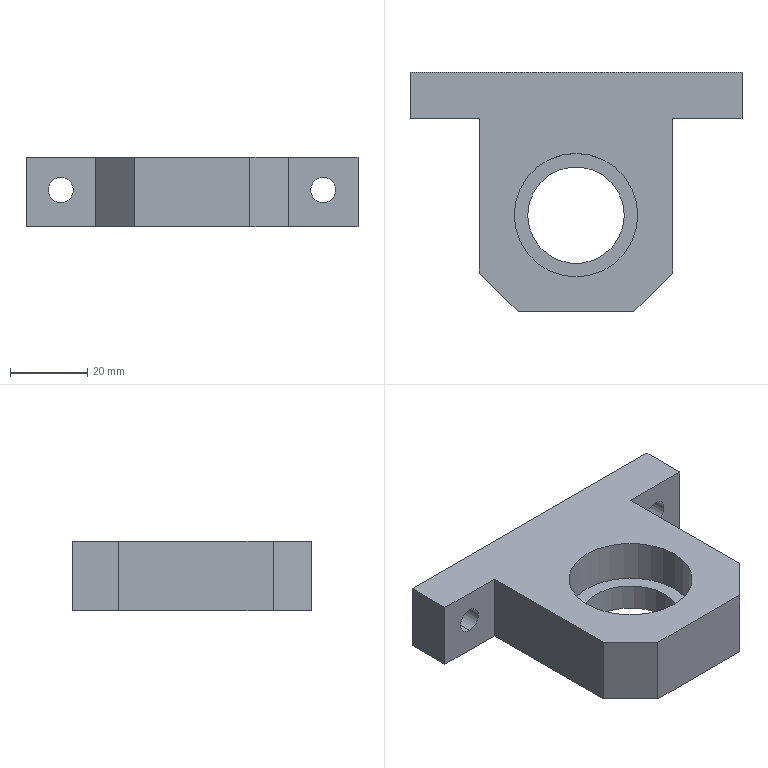Component | SolidWorks | --MA18S20041JR-SHuangGWBearingHousing1-1 | 1 solid | 21 faces | box 86 x 62 x 18 mm | volume 48697 mm3 | plane 13 | cylinder 8 | commonest cylinder face diameters 6.5 x4 25 x2 32 x2
build123d program:
from build123d import *

# Parameters (mm, degrees)
SKETCH1_W                  = 50
SKETCH1_H                  = 50
BOSS_EXTRUDE1_DEPTH        = 18
SKETCH2_W                  = 86
SKETCH2_H                  = 18
BOSS_EXTRUDE2_DEPTH        = 12
CHAMFER1_SIZE              = 10
SKETCH3_R                  = 16
CUT_EXTRUDE1_DEPTH         = 11
SKETCH4_R                  = 12.5
CUT_EXTRUDE2_DEPTH         = 86.118
F_6_5_6_5_DIAMETER_HOLE1_D = 6.5


with BuildPart() as part:
    # Sketch1 → Boss-Extrude1 (new body)
    with BuildSketch(Plane.XY):
        with Locations((25, 25)):
            Rectangle(SKETCH1_W, SKETCH1_H)
    extrude(amount=BOSS_EXTRUDE1_DEPTH)

    # Sketch2 → Boss-Extrude2 (add)
    with BuildSketch(Plane.XZ):
        with Locations((25, 9)):
            Rectangle(SKETCH2_W, SKETCH2_H)
    extrude(amount=BOSS_EXTRUDE2_DEPTH)

    # Chamfer1
    chamfer1_edges = [part.edges().sort_by_distance(p)[0] for p in [
        (0, 50, 9),
        (50, 50, 9),
    ]]
    chamfer(chamfer1_edges, length=CHAMFER1_SIZE)

    # Sketch3 → Cut-Extrude1 (cut)
    with BuildSketch(Plane.XY.offset(18)):
        with Locations((25, 25)):
            Circle(SKETCH3_R)
    extrude(amount=-CUT_EXTRUDE1_DEPTH, mode=Mode.SUBTRACT)

    # Sketch4 → Cut-Extrude2 (cut, through all)
    with BuildSketch(Plane.XY.offset(7)):
        with Locations((25, 25)):
            Circle(SKETCH4_R)
    extrude(amount=-CUT_EXTRUDE2_DEPTH, mode=Mode.SUBTRACT)

    # 6.5 _6.5_ Diameter Hole1 (through all)
    with Locations(Plane(origin=(0, 0, 0), x_dir=(-1, 0, 0), z_dir=(0, 1, 0))):
        with Locations((-59, 9.5), (9, 9.5)):
            Hole(F_6_5_6_5_DIAMETER_HOLE1_D / 2)


solid = part.part

# Placed as in the assembly
solid = solid.moved(Location((97.885, -8.301, 1), (0, 0, 180)))
STEP:
#1=COLOUR_RGB('',0.7922,0.8196,0.9333);
#2=FILL_AREA_STYLE_COLOUR('',#1);
#3=FILL_AREA_STYLE('',(#2));
#4=SURFACE_STYLE_FILL_AREA(#3);
#5=SURFACE_SIDE_STYLE('',(#4));
#6=SURFACE_STYLE_USAGE(.BOTH.,#5);
#7=PRESENTATION_STYLE_ASSIGNMENT((#6));
#8=CARTESIAN_POINT('',(1.531,0.1456,0.2854));
#9=VERTEX_POINT('',#8);
#10=CARTESIAN_POINT('',(1.531,0.1456,0.5413));
#11=VERTEX_POINT('',#10);
#12=CARTESIAN_POINT('',(1.531,0.1456,0.4134));
#13=DIRECTION('',(-0.,-1.,0.));
#14=DIRECTION('',(0.,0.,1.));
#15=AXIS2_PLACEMENT_3D('',#12,#13,#14);
#16=CIRCLE('',#15,0.128);
#17=EDGE_CURVE('',#9,#11,#16,.T.);
#18=ORIENTED_EDGE('',*,*,#17,.F.);
#19=CARTESIAN_POINT('',(1.531,-0.3268,0.2854));
#20=VERTEX_POINT('',#19);
#21=CARTESIAN_POINT('',(1.531,-0.3268,0.2854));
#22=DIRECTION('',(-0.,-1.,0.));
#23=VECTOR('',#22,39.37);
#24=LINE('',#21,#23);
#25=EDGE_CURVE('',#9,#20,#24,.T.);
#26=ORIENTED_EDGE('',*,*,#25,.T.);
#27=CARTESIAN_POINT('',(1.531,-0.3268,0.5413));
#28=VERTEX_POINT('',#27);
#29=CARTESIAN_POINT('',(1.531,-0.3268,0.4134));
#30=DIRECTION('',(-0.,-1.,0.));
#31=DIRECTION('',(0.,0.,1.));
#32=AXIS2_PLACEMENT_3D('',#29,#30,#31);
#33=CIRCLE('',#32,0.128);
#34=EDGE_CURVE('',#20,#28,#33,.T.);
#35=ORIENTED_EDGE('',*,*,#34,.T.);
#36=CARTESIAN_POINT('',(1.531,-0.3268,0.5413));
#37=DIRECTION('',(-0.,-1.,0.));
#38=VECTOR('',#37,39.37);
#39=LINE('',#36,#38);
#40=EDGE_CURVE('',#11,#28,#39,.T.);
#41=ORIENTED_EDGE('',*,*,#40,.F.);
#42=EDGE_LOOP('',(#18,#26,#35,#41));
#43=FACE_OUTER_BOUND('',#42,.T.);
#44=CARTESIAN_POINT('',(1.531,-0.3268,0.4134));
#45=DIRECTION('',(-0.,-1.,0.));
#46=DIRECTION('',(0.,0.,1.));
#47=AXIS2_PLACEMENT_3D('',#44,#45,#46);
#48=CYLINDRICAL_SURFACE('',#47,0.128);
#49=ADVANCED_FACE('',(#43),#48,.F.);
#50=CARTESIAN_POINT('',(4.208,0.1456,0.2854));
#51=VERTEX_POINT('',#50);
#52=CARTESIAN_POINT('',(4.208,0.1456,0.5413));
#53=VERTEX_POINT('',#52);
#54=CARTESIAN_POINT('',(4.208,0.1456,0.4134));
#55=DIRECTION('',(-0.,-1.,0.));
#56=DIRECTION('',(0.,0.,1.));
#57=AXIS2_PLACEMENT_3D('',#54,#55,#56);
#58=CIRCLE('',#57,0.128);
#59=EDGE_CURVE('',#51,#53,#58,.T.);
#60=ORIENTED_EDGE('',*,*,#59,.F.);
#61=CARTESIAN_POINT('',(4.208,-0.3268,0.2854));
#62=VERTEX_POINT('',#61);
#63=CARTESIAN_POINT('',(4.208,-0.3268,0.2854));
#64=DIRECTION('',(-0.,-1.,0.));
#65=VECTOR('',#64,39.37);
#66=LINE('',#63,#65);
#67=EDGE_CURVE('',#51,#62,#66,.T.);
#68=ORIENTED_EDGE('',*,*,#67,.T.);
#69=CARTESIAN_POINT('',(4.208,-0.3268,0.5413));
#70=VERTEX_POINT('',#69);
#71=CARTESIAN_POINT('',(4.208,-0.3268,0.4134));
#72=DIRECTION('',(-0.,-1.,0.));
#73=DIRECTION('',(0.,0.,1.));
#74=AXIS2_PLACEMENT_3D('',#71,#72,#73);
#75=CIRCLE('',#74,0.128);
#76=EDGE_CURVE('',#62,#70,#75,.T.);
#77=ORIENTED_EDGE('',*,*,#76,.T.);
#78=CARTESIAN_POINT('',(4.208,-0.3268,0.5413));
#79=DIRECTION('',(-0.,-1.,0.));
#80=VECTOR('',#79,39.37);
#81=LINE('',#78,#80);
#82=EDGE_CURVE('',#53,#70,#81,.T.);
#83=ORIENTED_EDGE('',*,*,#82,.F.);
#84=EDGE_LOOP('',(#60,#68,#77,#83));
#85=FACE_OUTER_BOUND('',#84,.T.);
#86=CARTESIAN_POINT('',(4.208,-0.3268,0.4134));
#87=DIRECTION('',(-0.,-1.,0.));
#88=DIRECTION('',(0.,0.,1.));
#89=AXIS2_PLACEMENT_3D('',#86,#87,#88);
#90=CYLINDRICAL_SURFACE('',#89,0.128);
#91=ADVANCED_FACE('',(#85),#90,.F.);
#92=CARTESIAN_POINT('',(2.377,-1.311,0.03937));
#93=VERTEX_POINT('',#92);
#94=CARTESIAN_POINT('',(3.362,-1.311,0.03937));
#95=VERTEX_POINT('',#94);
#96=CARTESIAN_POINT('',(2.869,-1.311,0.03937));
#97=DIRECTION('',(-0.,-0.,-1.));
#98=DIRECTION('',(1.,0.,-0.));
#99=AXIS2_PLACEMENT_3D('',#96,#97,#98);
#100=CIRCLE('',#99,0.4921);
#101=EDGE_CURVE('',#93,#95,#100,.T.);
#102=ORIENTED_EDGE('',*,*,#101,.T.);
#103=CARTESIAN_POINT('',(3.362,-1.311,0.315));
#104=VERTEX_POINT('',#103);
#105=CARTESIAN_POINT('',(3.362,-1.311,0.03937));
#106=DIRECTION('',(0.,0.,1.));
#107=VECTOR('',#106,39.37);
#108=LINE('',#105,#107);
#109=EDGE_CURVE('',#95,#104,#108,.T.);
#110=ORIENTED_EDGE('',*,*,#109,.T.);
#111=CARTESIAN_POINT('',(2.377,-1.311,0.315));
#112=VERTEX_POINT('',#111);
#113=CARTESIAN_POINT('',(2.869,-1.311,0.315));
#114=DIRECTION('',(0.,0.,1.));
#115=DIRECTION('',(-1.,0.,0.));
#116=AXIS2_PLACEMENT_3D('',#113,#114,#115);
#117=CIRCLE('',#116,0.4921);
#118=EDGE_CURVE('',#104,#112,#117,.T.);
#119=ORIENTED_EDGE('',*,*,#118,.T.);
#120=CARTESIAN_POINT('',(2.377,-1.311,0.03937));
#121=DIRECTION('',(0.,0.,1.));
#122=VECTOR('',#121,39.37);
#123=LINE('',#120,#122);
#124=EDGE_CURVE('',#93,#112,#123,.T.);
#125=ORIENTED_EDGE('',*,*,#124,.F.);
#126=EDGE_LOOP('',(#102,#110,#119,#125));
#127=FACE_OUTER_BOUND('',#126,.T.);
#128=CARTESIAN_POINT('',(2.869,-1.311,0.03937));
#129=DIRECTION('',(0.,0.,1.));
#130=DIRECTION('',(-1.,0.,0.));
#131=AXIS2_PLACEMENT_3D('',#128,#129,#130);
#132=CYLINDRICAL_SURFACE('',#131,0.4921);
#133=ADVANCED_FACE('',(#127),#132,.F.);
#134=CARTESIAN_POINT('',(3.499,-1.311,0.315));
#135=VERTEX_POINT('',#134);
#136=CARTESIAN_POINT('',(2.24,-1.311,0.315));
#137=VERTEX_POINT('',#136);
#138=CARTESIAN_POINT('',(2.869,-1.311,0.315));
#139=DIRECTION('',(0.,0.,1.));
#140=DIRECTION('',(-1.,0.,0.));
#141=AXIS2_PLACEMENT_3D('',#138,#139,#140);
#142=CIRCLE('',#141,0.6299);
#143=EDGE_CURVE('',#135,#137,#142,.T.);
#144=ORIENTED_EDGE('',*,*,#143,.F.);
#145=CARTESIAN_POINT('',(3.499,-1.311,0.748));
#146=VERTEX_POINT('',#145);
#147=CARTESIAN_POINT('',(3.499,-1.311,0.315));
#148=DIRECTION('',(0.,0.,1.));
#149=VECTOR('',#148,39.37);
#150=LINE('',#147,#149);
#151=EDGE_CURVE('',#135,#146,#150,.T.);
#152=ORIENTED_EDGE('',*,*,#151,.T.);
#153=CARTESIAN_POINT('',(2.24,-1.311,0.748));
#154=VERTEX_POINT('',#153);
#155=CARTESIAN_POINT('',(2.869,-1.311,0.748));
#156=DIRECTION('',(0.,0.,1.));
#157=DIRECTION('',(-1.,0.,0.));
#158=AXIS2_PLACEMENT_3D('',#155,#156,#157);
#159=CIRCLE('',#158,0.6299);
#160=EDGE_CURVE('',#146,#154,#159,.T.);
#161=ORIENTED_EDGE('',*,*,#160,.T.);
#162=CARTESIAN_POINT('',(2.24,-1.311,0.315));
#163=DIRECTION('',(0.,0.,1.));
#164=VECTOR('',#163,39.37);
#165=LINE('',#162,#164);
#166=EDGE_CURVE('',#137,#154,#165,.T.);
#167=ORIENTED_EDGE('',*,*,#166,.F.);
#168=EDGE_LOOP('',(#144,#152,#161,#167));
#169=FACE_OUTER_BOUND('',#168,.T.);
#170=CARTESIAN_POINT('',(2.869,-1.311,0.315));
#171=DIRECTION('',(0.,0.,1.));
#172=DIRECTION('',(-1.,0.,0.));
#173=AXIS2_PLACEMENT_3D('',#170,#171,#172);
#174=CYLINDRICAL_SURFACE('',#173,0.6299);
#175=ADVANCED_FACE('',(#169),#174,.F.);
#176=CARTESIAN_POINT('',(1.885,-0.3268,0.748));
#177=VERTEX_POINT('',#176);
#178=CARTESIAN_POINT('',(1.885,-0.3268,0.03937));
#179=VERTEX_POINT('',#178);
#180=CARTESIAN_POINT('',(1.885,-0.3268,0.748));
#181=DIRECTION('',(-0.,-0.,-1.));
#182=VECTOR('',#181,39.37);
#183=LINE('',#180,#182);
#184=EDGE_CURVE('',#177,#179,#183,.T.);
#185=ORIENTED_EDGE('',*,*,#184,.F.);
#186=CARTESIAN_POINT('',(1.177,-0.3268,0.748));
#187=VERTEX_POINT('',#186);
#188=CARTESIAN_POINT('',(4.562,-0.3268,0.748));
#189=DIRECTION('',(1.,0.,-0.));
#190=VECTOR('',#189,39.37);
#191=LINE('',#188,#190);
#192=EDGE_CURVE('',#187,#177,#191,.T.);
#193=ORIENTED_EDGE('',*,*,#192,.F.);
#194=CARTESIAN_POINT('',(1.177,-0.3268,0.03937));
#195=VERTEX_POINT('',#194);
#196=CARTESIAN_POINT('',(1.177,-0.3268,0.748));
#197=DIRECTION('',(0.,0.,1.));
#198=VECTOR('',#197,39.37);
#199=LINE('',#196,#198);
#200=EDGE_CURVE('',#195,#187,#199,.T.);
#201=ORIENTED_EDGE('',*,*,#200,.F.);
#202=CARTESIAN_POINT('',(4.562,-0.3268,0.03937));
#203=DIRECTION('',(-1.,-0.,0.));
#204=VECTOR('',#203,39.37);
#205=LINE('',#202,#204);
#206=EDGE_CURVE('',#179,#195,#205,.T.);
#207=ORIENTED_EDGE('',*,*,#206,.F.);
#208=EDGE_LOOP('',(#185,#193,#201,#207));
#209=FACE_OUTER_BOUND('',#208,.T.);
#210=CARTESIAN_POINT('',(1.531,-0.3268,0.4134));
#211=DIRECTION('',(-0.,-1.,0.));
#212=DIRECTION('',(0.,0.,1.));
#213=AXIS2_PLACEMENT_3D('',#210,#211,#212);
#214=CIRCLE('',#213,0.128);
#215=EDGE_CURVE('',#28,#20,#214,.T.);
#216=ORIENTED_EDGE('',*,*,#215,.F.);
#217=ORIENTED_EDGE('',*,*,#34,.F.);
#218=EDGE_LOOP('',(#216,#217));
#219=FACE_BOUND('',#218,.T.);
#220=CARTESIAN_POINT('',(4.562,-0.3268,0.03937));
#221=DIRECTION('',(0.,1.,-0.));
#222=DIRECTION('',(-0.,-0.,-1.));
#223=AXIS2_PLACEMENT_3D('',#220,#221,#222);
#224=PLANE('',#223);
#225=ADVANCED_FACE('',(#209,#219),#224,.F.);
#226=CARTESIAN_POINT('',(3.854,-1.902,0.748));
#227=VERTEX_POINT('',#226);
#228=CARTESIAN_POINT('',(3.854,-0.3268,0.748));
#229=VERTEX_POINT('',#228);
#230=CARTESIAN_POINT('',(3.854,-0.3268,0.748));
#231=DIRECTION('',(-0.,1.,-0.));
#232=VECTOR('',#231,39.37);
#233=LINE('',#230,#232);
#234=EDGE_CURVE('',#227,#229,#233,.T.);
#235=ORIENTED_EDGE('',*,*,#234,.F.);
#236=CARTESIAN_POINT('',(3.854,-1.902,0.03937));
#237=VERTEX_POINT('',#236);
#238=CARTESIAN_POINT('',(3.854,-1.902,0.748));
#239=DIRECTION('',(-0.,-0.,-1.));
#240=VECTOR('',#239,39.37);
#241=LINE('',#238,#240);
#242=EDGE_CURVE('',#227,#237,#241,.T.);
#243=ORIENTED_EDGE('',*,*,#242,.T.);
#244=CARTESIAN_POINT('',(3.854,-0.3268,0.03937));
#245=VERTEX_POINT('',#244);
#246=CARTESIAN_POINT('',(3.854,-0.3268,0.03937));
#247=DIRECTION('',(-0.,1.,-0.));
#248=VECTOR('',#247,39.37);
#249=LINE('',#246,#248);
#250=EDGE_CURVE('',#237,#245,#249,.T.);
#251=ORIENTED_EDGE('',*,*,#250,.T.);
#252=CARTESIAN_POINT('',(3.854,-0.3268,0.748));
#253=DIRECTION('',(-0.,-0.,-1.));
#254=VECTOR('',#253,39.37);
#255=LINE('',#252,#254);
#256=EDGE_CURVE('',#229,#245,#255,.T.);
#257=ORIENTED_EDGE('',*,*,#256,.F.);
#258=EDGE_LOOP('',(#235,#243,#251,#257));
#259=FACE_OUTER_BOUND('',#258,.T.);
#260=CARTESIAN_POINT('',(3.854,-0.3268,0.748));
#261=DIRECTION('',(-1.,-0.,0.));
#262=DIRECTION('',(0.,-1.,0.));
#263=AXIS2_PLACEMENT_3D('',#260,#261,#262);
#264=PLANE('',#263);
#265=ADVANCED_FACE('',(#259),#264,.F.);
#266=CARTESIAN_POINT('',(1.885,-1.902,0.03937));
#267=VERTEX_POINT('',#266);
#268=CARTESIAN_POINT('',(1.885,-0.3268,0.03937));
#269=DIRECTION('',(0.,-1.,0.));
#270=VECTOR('',#269,39.37);
#271=LINE('',#268,#270);
#272=EDGE_CURVE('',#179,#267,#271,.T.);
#273=ORIENTED_EDGE('',*,*,#272,.T.);
#274=CARTESIAN_POINT('',(1.885,-1.902,0.748));
#275=VERTEX_POINT('',#274);
#276=CARTESIAN_POINT('',(1.885,-1.902,0.748));
#277=DIRECTION('',(0.,0.,1.));
#278=VECTOR('',#277,39.37);
#279=LINE('',#276,#278);
#280=EDGE_CURVE('',#267,#275,#279,.T.);
#281=ORIENTED_EDGE('',*,*,#280,.T.);
#282=CARTESIAN_POINT('',(1.885,-0.3268,0.748));
#283=DIRECTION('',(0.,-1.,0.));
#284=VECTOR('',#283,39.37);
#285=LINE('',#282,#284);
#286=EDGE_CURVE('',#177,#275,#285,.T.);
#287=ORIENTED_EDGE('',*,*,#286,.F.);
#288=ORIENTED_EDGE('',*,*,#184,.T.);
#289=EDGE_LOOP('',(#273,#281,#287,#288));
#290=FACE_OUTER_BOUND('',#289,.T.);
#291=CARTESIAN_POINT('',(1.885,-0.3268,0.748));
#292=DIRECTION('',(1.,0.,-0.));
#293=DIRECTION('',(-0.,1.,-0.));
#294=AXIS2_PLACEMENT_3D('',#291,#292,#293);
#295=PLANE('',#294);
#296=ADVANCED_FACE('',(#290),#295,.F.);
#297=CARTESIAN_POINT('',(2.279,-2.295,0.03937));
#298=VERTEX_POINT('',#297);
#299=CARTESIAN_POINT('',(3.46,-2.295,0.03937));
#300=VERTEX_POINT('',#299);
#301=CARTESIAN_POINT('',(3.854,-2.295,0.03937));
#302=DIRECTION('',(1.,0.,-0.));
#303=VECTOR('',#302,39.37);
#304=LINE('',#301,#303);
#305=EDGE_CURVE('',#298,#300,#304,.T.);
#306=ORIENTED_EDGE('',*,*,#305,.T.);
#307=CARTESIAN_POINT('',(3.46,-2.295,0.748));
#308=VERTEX_POINT('',#307);
#309=CARTESIAN_POINT('',(3.46,-2.295,0.748));
#310=DIRECTION('',(0.,0.,1.));
#311=VECTOR('',#310,39.37);
#312=LINE('',#309,#311);
#313=EDGE_CURVE('',#300,#308,#312,.T.);
#314=ORIENTED_EDGE('',*,*,#313,.T.);
#315=CARTESIAN_POINT('',(2.279,-2.295,0.748));
#316=VERTEX_POINT('',#315);
#317=CARTESIAN_POINT('',(3.854,-2.295,0.748));
#318=DIRECTION('',(1.,0.,-0.));
#319=VECTOR('',#318,39.37);
#320=LINE('',#317,#319);
#321=EDGE_CURVE('',#316,#308,#320,.T.);
#322=ORIENTED_EDGE('',*,*,#321,.F.);
#323=CARTESIAN_POINT('',(2.279,-2.295,0.748));
#324=DIRECTION('',(-0.,-0.,-1.));
#325=VECTOR('',#324,39.37);
#326=LINE('',#323,#325);
#327=EDGE_CURVE('',#316,#298,#326,.T.);
#328=ORIENTED_EDGE('',*,*,#327,.T.);
#329=EDGE_LOOP('',(#306,#314,#322,#328));
#330=FACE_OUTER_BOUND('',#329,.T.);
#331=CARTESIAN_POINT('',(3.854,-2.295,0.748));
#332=DIRECTION('',(0.,1.,-0.));
#333=DIRECTION('',(-0.,-0.,-1.));
#334=AXIS2_PLACEMENT_3D('',#331,#332,#333);
#335=PLANE('',#334);
#336=ADVANCED_FACE('',(#330),#335,.F.);
#337=CARTESIAN_POINT('',(2.869,-1.311,0.748));
#338=DIRECTION('',(0.,0.,1.));
#339=DIRECTION('',(-1.,0.,0.));
#340=AXIS2_PLACEMENT_3D('',#337,#338,#339);
#341=CIRCLE('',#340,0.6299);
#342=EDGE_CURVE('',#154,#146,#341,.T.);
#343=ORIENTED_EDGE('',*,*,#342,.F.);
#344=ORIENTED_EDGE('',*,*,#160,.F.);
#345=EDGE_LOOP('',(#343,#344));
#346=FACE_BOUND('',#345,.T.);
#347=ORIENTED_EDGE('',*,*,#321,.T.);
#348=CARTESIAN_POINT('',(3.854,-1.902,0.748));
#349=DIRECTION('',(0.7071,0.7071,-0.));
#350=VECTOR('',#349,39.37);
#351=LINE('',#348,#350);
#352=EDGE_CURVE('',#308,#227,#351,.T.);
#353=ORIENTED_EDGE('',*,*,#352,.T.);
#354=ORIENTED_EDGE('',*,*,#234,.T.);
#355=CARTESIAN_POINT('',(4.562,-0.3268,0.748));
#356=VERTEX_POINT('',#355);
#357=CARTESIAN_POINT('',(4.562,-0.3268,0.748));
#358=DIRECTION('',(1.,0.,-0.));
#359=VECTOR('',#358,39.37);
#360=LINE('',#357,#359);
#361=EDGE_CURVE('',#229,#356,#360,.T.);
#362=ORIENTED_EDGE('',*,*,#361,.T.);
#363=CARTESIAN_POINT('',(4.562,0.1456,0.748));
#364=VERTEX_POINT('',#363);
#365=CARTESIAN_POINT('',(4.562,0.1456,0.748));
#366=DIRECTION('',(-0.,-1.,0.));
#367=VECTOR('',#366,39.37);
#368=LINE('',#365,#367);
#369=EDGE_CURVE('',#364,#356,#368,.T.);
#370=ORIENTED_EDGE('',*,*,#369,.F.);
#371=CARTESIAN_POINT('',(1.177,0.1456,0.748));
#372=VERTEX_POINT('',#371);
#373=CARTESIAN_POINT('',(4.562,0.1456,0.748));
#374=DIRECTION('',(1.,0.,-0.));
#375=VECTOR('',#374,39.37);
#376=LINE('',#373,#375);
#377=EDGE_CURVE('',#372,#364,#376,.T.);
#378=ORIENTED_EDGE('',*,*,#377,.F.);
#379=CARTESIAN_POINT('',(1.177,0.1456,0.748));
#380=DIRECTION('',(-0.,-1.,0.));
#381=VECTOR('',#380,39.37);
#382=LINE('',#379,#381);
#383=EDGE_CURVE('',#372,#187,#382,.T.);
#384=ORIENTED_EDGE('',*,*,#383,.T.);
#385=ORIENTED_EDGE('',*,*,#192,.T.);
#386=ORIENTED_EDGE('',*,*,#286,.T.);
#387=CARTESIAN_POINT('',(2.279,-2.295,0.748));
#388=DIRECTION('',(0.7071,-0.7071,0.));
#389=VECTOR('',#388,39.37);
#390=LINE('',#387,#389);
#391=EDGE_CURVE('',#275,#316,#390,.T.);
#392=ORIENTED_EDGE('',*,*,#391,.T.);
#393=EDGE_LOOP('',(#347,#353,#354,#362,#370,#378,#384,#385,#386,#392));
#394=FACE_OUTER_BOUND('',#393,.T.);
#395=CARTESIAN_POINT('',(3.854,-2.295,0.748));
#396=DIRECTION('',(-0.,-0.,-1.));
#397=DIRECTION('',(1.,0.,-0.));
#398=AXIS2_PLACEMENT_3D('',#395,#396,#397);
#399=PLANE('',#398);
#400=ADVANCED_FACE('',(#346,#394),#399,.F.);
#401=ORIENTED_EDGE('',*,*,#101,.F.);
#402=CARTESIAN_POINT('',(2.869,-1.311,0.03937));
#403=DIRECTION('',(-0.,-0.,-1.));
#404=DIRECTION('',(1.,0.,-0.));
#405=AXIS2_PLACEMENT_3D('',#402,#403,#404);
#406=CIRCLE('',#405,0.4921);
#407=EDGE_CURVE('',#95,#93,#406,.T.);
#408=ORIENTED_EDGE('',*,*,#407,.F.);
#409=EDGE_LOOP('',(#401,#408));
#410=FACE_BOUND('',#409,.T.);
#411=ORIENTED_EDGE('',*,*,#250,.F.);
#412=CARTESIAN_POINT('',(3.657,-2.098,0.03937));
#413=DIRECTION('',(-0.7071,-0.7071,0.));
#414=VECTOR('',#413,39.37);
#415=LINE('',#412,#414);
#416=EDGE_CURVE('',#237,#300,#415,.T.);
#417=ORIENTED_EDGE('',*,*,#416,.T.);
#418=ORIENTED_EDGE('',*,*,#305,.F.);
#419=CARTESIAN_POINT('',(3.066,-3.083,0.03937));
#420=DIRECTION('',(-0.7071,0.7071,-0.));
#421=VECTOR('',#420,39.37);
#422=LINE('',#419,#421);
#423=EDGE_CURVE('',#298,#267,#422,.T.);
#424=ORIENTED_EDGE('',*,*,#423,.T.);
#425=ORIENTED_EDGE('',*,*,#272,.F.);
#426=ORIENTED_EDGE('',*,*,#206,.T.);
#427=CARTESIAN_POINT('',(1.177,0.1456,0.03937));
#428=VERTEX_POINT('',#427);
#429=CARTESIAN_POINT('',(1.177,0.1456,0.03937));
#430=DIRECTION('',(-0.,-1.,0.));
#431=VECTOR('',#430,39.37);
#432=LINE('',#429,#431);
#433=EDGE_CURVE('',#428,#195,#432,.T.);
#434=ORIENTED_EDGE('',*,*,#433,.F.);
#435=CARTESIAN_POINT('',(4.562,0.1456,0.03937));
#436=VERTEX_POINT('',#435);
#437=CARTESIAN_POINT('',(4.562,0.1456,0.03937));
#438=DIRECTION('',(-1.,-0.,0.));
#439=VECTOR('',#438,39.37);
#440=LINE('',#437,#439);
#441=EDGE_CURVE('',#436,#428,#440,.T.);
#442=ORIENTED_EDGE('',*,*,#441,.F.);
#443=CARTESIAN_POINT('',(4.562,-0.3268,0.03937));
#444=VERTEX_POINT('',#443);
#445=CARTESIAN_POINT('',(4.562,0.1456,0.03937));
#446=DIRECTION('',(-0.,-1.,0.));
#447=VECTOR('',#446,39.37);
#448=LINE('',#445,#447);
#449=EDGE_CURVE('',#436,#444,#448,.T.);
#450=ORIENTED_EDGE('',*,*,#449,.T.);
#451=CARTESIAN_POINT('',(4.562,-0.3268,0.03937));
#452=DIRECTION('',(-1.,-0.,0.));
#453=VECTOR('',#452,39.37);
#454=LINE('',#451,#453);
#455=EDGE_CURVE('',#444,#245,#454,.T.);
#456=ORIENTED_EDGE('',*,*,#455,.T.);
#457=EDGE_LOOP('',(#411,#417,#418,#424,#425,#426,#434,#442,#450,#456));
#458=FACE_OUTER_BOUND('',#457,.T.);
#459=CARTESIAN_POINT('',(3.854,-2.295,0.03937));
#460=DIRECTION('',(-0.,-0.,-1.));
#461=DIRECTION('',(1.,0.,-0.));
#462=AXIS2_PLACEMENT_3D('',#459,#460,#461);
#463=PLANE('',#462);
#464=ADVANCED_FACE('',(#410,#458),#463,.T.);
#465=CARTESIAN_POINT('',(4.208,-0.3268,0.4134));
#466=DIRECTION('',(-0.,-1.,0.));
#467=DIRECTION('',(0.,0.,1.));
#468=AXIS2_PLACEMENT_3D('',#465,#466,#467);
#469=CIRCLE('',#468,0.128);
#470=EDGE_CURVE('',#70,#62,#469,.T.);
#471=ORIENTED_EDGE('',*,*,#470,.F.);
#472=ORIENTED_EDGE('',*,*,#76,.F.);
#473=EDGE_LOOP('',(#471,#472));
#474=FACE_BOUND('',#473,.T.);
#475=ORIENTED_EDGE('',*,*,#361,.F.);
#476=ORIENTED_EDGE('',*,*,#256,.T.);
#477=ORIENTED_EDGE('',*,*,#455,.F.);
#478=CARTESIAN_POINT('',(4.562,-0.3268,0.748));
#479=DIRECTION('',(-0.,-0.,-1.));
#480=VECTOR('',#479,39.37);
#481=LINE('',#478,#480);
#482=EDGE_CURVE('',#356,#444,#481,.T.);
#483=ORIENTED_EDGE('',*,*,#482,.F.);
#484=EDGE_LOOP('',(#475,#476,#477,#483));
#485=FACE_OUTER_BOUND('',#484,.T.);
#486=CARTESIAN_POINT('',(4.562,-0.3268,0.03937));
#487=DIRECTION('',(0.,1.,-0.));
#488=DIRECTION('',(-0.,-0.,-1.));
#489=AXIS2_PLACEMENT_3D('',#486,#487,#488);
#490=PLANE('',#489);
#491=ADVANCED_FACE('',(#474,#485),#490,.F.);
#492=ORIENTED_EDGE('',*,*,#482,.T.);
#493=ORIENTED_EDGE('',*,*,#449,.F.);
#494=CARTESIAN_POINT('',(4.562,0.1456,0.748));
#495=DIRECTION('',(-0.,-0.,-1.));
#496=VECTOR('',#495,39.37);
#497=LINE('',#494,#496);
#498=EDGE_CURVE('',#364,#436,#497,.T.);
#499=ORIENTED_EDGE('',*,*,#498,.F.);
#500=ORIENTED_EDGE('',*,*,#369,.T.);
#501=EDGE_LOOP('',(#492,#493,#499,#500));
#502=FACE_OUTER_BOUND('',#501,.T.);
#503=CARTESIAN_POINT('',(4.562,0.1456,0.748));
#504=DIRECTION('',(-1.,-0.,0.));
#505=DIRECTION('',(-0.,-0.,-1.));
#506=AXIS2_PLACEMENT_3D('',#503,#504,#505);
#507=PLANE('',#506);
#508=ADVANCED_FACE('',(#502),#507,.F.);
#509=ORIENTED_EDGE('',*,*,#200,.T.);
#510=ORIENTED_EDGE('',*,*,#383,.F.);
#511=CARTESIAN_POINT('',(1.177,0.1456,0.748));
#512=DIRECTION('',(0.,0.,1.));
#513=VECTOR('',#512,39.37);
#514=LINE('',#511,#513);
#515=EDGE_CURVE('',#428,#372,#514,.T.);
#516=ORIENTED_EDGE('',*,*,#515,.F.);
#517=ORIENTED_EDGE('',*,*,#433,.T.);
#518=EDGE_LOOP('',(#509,#510,#516,#517));
#519=FACE_OUTER_BOUND('',#518,.T.);
#520=CARTESIAN_POINT('',(1.177,0.1456,0.748));
#521=DIRECTION('',(1.,0.,-0.));
#522=DIRECTION('',(0.,0.,1.));
#523=AXIS2_PLACEMENT_3D('',#520,#521,#522);
#524=PLANE('',#523);
#525=ADVANCED_FACE('',(#519),#524,.F.);
#526=CARTESIAN_POINT('',(1.531,0.1456,0.4134));
#527=DIRECTION('',(-0.,-1.,0.));
#528=DIRECTION('',(0.,0.,1.));
#529=AXIS2_PLACEMENT_3D('',#526,#527,#528);
#530=CIRCLE('',#529,0.128);
#531=EDGE_CURVE('',#11,#9,#530,.T.);
#532=ORIENTED_EDGE('',*,*,#531,.T.);
#533=ORIENTED_EDGE('',*,*,#17,.T.);
#534=EDGE_LOOP('',(#532,#533));
#535=FACE_BOUND('',#534,.T.);
#536=CARTESIAN_POINT('',(4.208,0.1456,0.4134));
#537=DIRECTION('',(-0.,-1.,0.));
#538=DIRECTION('',(0.,0.,1.));
#539=AXIS2_PLACEMENT_3D('',#536,#537,#538);
#540=CIRCLE('',#539,0.128);
#541=EDGE_CURVE('',#53,#51,#540,.T.);
#542=ORIENTED_EDGE('',*,*,#541,.T.);
#543=ORIENTED_EDGE('',*,*,#59,.T.);
#544=EDGE_LOOP('',(#542,#543));
#545=FACE_BOUND('',#544,.T.);
#546=ORIENTED_EDGE('',*,*,#498,.T.);
#547=ORIENTED_EDGE('',*,*,#441,.T.);
#548=ORIENTED_EDGE('',*,*,#515,.T.);
#549=ORIENTED_EDGE('',*,*,#377,.T.);
#550=EDGE_LOOP('',(#546,#547,#548,#549));
#551=FACE_OUTER_BOUND('',#550,.T.);
#552=CARTESIAN_POINT('',(4.562,0.1456,0.03937));
#553=DIRECTION('',(0.,1.,-0.));
#554=DIRECTION('',(-0.,-0.,-1.));
#555=AXIS2_PLACEMENT_3D('',#552,#553,#554);
#556=PLANE('',#555);
#557=ADVANCED_FACE('',(#535,#545,#551),#556,.T.);
#558=ORIENTED_EDGE('',*,*,#352,.F.);
#559=ORIENTED_EDGE('',*,*,#313,.F.);
#560=ORIENTED_EDGE('',*,*,#416,.F.);
#561=ORIENTED_EDGE('',*,*,#242,.F.);
#562=EDGE_LOOP('',(#558,#559,#560,#561));
#563=FACE_OUTER_BOUND('',#562,.T.);
#564=CARTESIAN_POINT('',(3.854,-1.902,0.748));
#565=DIRECTION('',(-0.7071,0.7071,-0.));
#566=DIRECTION('',(-0.7071,-0.7071,0.));
#567=AXIS2_PLACEMENT_3D('',#564,#565,#566);
#568=PLANE('',#567);
#569=ADVANCED_FACE('',(#563),#568,.F.);
#570=ORIENTED_EDGE('',*,*,#391,.F.);
#571=ORIENTED_EDGE('',*,*,#280,.F.);
#572=ORIENTED_EDGE('',*,*,#423,.F.);
#573=ORIENTED_EDGE('',*,*,#327,.F.);
#574=EDGE_LOOP('',(#570,#571,#572,#573));
#575=FACE_OUTER_BOUND('',#574,.T.);
#576=CARTESIAN_POINT('',(2.279,-2.295,0.748));
#577=DIRECTION('',(0.7071,0.7071,-0.));
#578=DIRECTION('',(-0.7071,0.7071,-0.));
#579=AXIS2_PLACEMENT_3D('',#576,#577,#578);
#580=PLANE('',#579);
#581=ADVANCED_FACE('',(#575),#580,.F.);
#582=ORIENTED_EDGE('',*,*,#151,.F.);
#583=CARTESIAN_POINT('',(2.869,-1.311,0.315));
#584=DIRECTION('',(0.,0.,1.));
#585=DIRECTION('',(-1.,0.,0.));
#586=AXIS2_PLACEMENT_3D('',#583,#584,#585);
#587=CIRCLE('',#586,0.6299);
#588=EDGE_CURVE('',#137,#135,#587,.T.);
#589=ORIENTED_EDGE('',*,*,#588,.F.);
#590=ORIENTED_EDGE('',*,*,#166,.T.);
#591=ORIENTED_EDGE('',*,*,#342,.T.);
#592=EDGE_LOOP('',(#582,#589,#590,#591));
#593=FACE_OUTER_BOUND('',#592,.T.);
#594=CARTESIAN_POINT('',(2.869,-1.311,0.315));
#595=DIRECTION('',(0.,0.,1.));
#596=DIRECTION('',(-1.,0.,0.));
#597=AXIS2_PLACEMENT_3D('',#594,#595,#596);
#598=CYLINDRICAL_SURFACE('',#597,0.6299);
#599=ADVANCED_FACE('',(#593),#598,.F.);
#600=CARTESIAN_POINT('',(2.869,-1.311,0.315));
#601=DIRECTION('',(0.,0.,1.));
#602=DIRECTION('',(-1.,0.,0.));
#603=AXIS2_PLACEMENT_3D('',#600,#601,#602);
#604=CIRCLE('',#603,0.4921);
#605=EDGE_CURVE('',#112,#104,#604,.T.);
#606=ORIENTED_EDGE('',*,*,#605,.F.);
#607=ORIENTED_EDGE('',*,*,#118,.F.);
#608=EDGE_LOOP('',(#606,#607));
#609=FACE_BOUND('',#608,.T.);
#610=ORIENTED_EDGE('',*,*,#588,.T.);
#611=ORIENTED_EDGE('',*,*,#143,.T.);
#612=EDGE_LOOP('',(#610,#611));
#613=FACE_OUTER_BOUND('',#612,.T.);
#614=CARTESIAN_POINT('',(2.869,-1.311,0.315));
#615=DIRECTION('',(0.,0.,1.));
#616=DIRECTION('',(-1.,-0.,0.));
#617=AXIS2_PLACEMENT_3D('',#614,#615,#616);
#618=PLANE('',#617);
#619=ADVANCED_FACE('',(#609,#613),#618,.T.);
#620=ORIENTED_EDGE('',*,*,#109,.F.);
#621=ORIENTED_EDGE('',*,*,#407,.T.);
#622=ORIENTED_EDGE('',*,*,#124,.T.);
#623=ORIENTED_EDGE('',*,*,#605,.T.);
#624=EDGE_LOOP('',(#620,#621,#622,#623));
#625=FACE_OUTER_BOUND('',#624,.T.);
#626=CARTESIAN_POINT('',(2.869,-1.311,0.03937));
#627=DIRECTION('',(0.,0.,1.));
#628=DIRECTION('',(-1.,0.,0.));
#629=AXIS2_PLACEMENT_3D('',#626,#627,#628);
#630=CYLINDRICAL_SURFACE('',#629,0.4921);
#631=ADVANCED_FACE('',(#625),#630,.F.);
#632=ORIENTED_EDGE('',*,*,#67,.F.);
#633=ORIENTED_EDGE('',*,*,#541,.F.);
#634=ORIENTED_EDGE('',*,*,#82,.T.);
#635=ORIENTED_EDGE('',*,*,#470,.T.);
#636=EDGE_LOOP('',(#632,#633,#634,#635));
#637=FACE_OUTER_BOUND('',#636,.T.);
#638=CARTESIAN_POINT('',(4.208,-0.3268,0.4134));
#639=DIRECTION('',(-0.,-1.,0.));
#640=DIRECTION('',(0.,0.,1.));
#641=AXIS2_PLACEMENT_3D('',#638,#639,#640);
#642=CYLINDRICAL_SURFACE('',#641,0.128);
#643=ADVANCED_FACE('',(#637),#642,.F.);
#644=ORIENTED_EDGE('',*,*,#25,.F.);
#645=ORIENTED_EDGE('',*,*,#531,.F.);
#646=ORIENTED_EDGE('',*,*,#40,.T.);
#647=ORIENTED_EDGE('',*,*,#215,.T.);
#648=EDGE_LOOP('',(#644,#645,#646,#647));
#649=FACE_OUTER_BOUND('',#648,.T.);
#650=CARTESIAN_POINT('',(1.531,-0.3268,0.4134));
#651=DIRECTION('',(-0.,-1.,0.));
#652=DIRECTION('',(0.,0.,1.));
#653=AXIS2_PLACEMENT_3D('',#650,#651,#652);
#654=CYLINDRICAL_SURFACE('',#653,0.128);
#655=ADVANCED_FACE('',(#649),#654,.F.);
#656=CLOSED_SHELL('',(#49,#91,#133,#175,#225,#265,#296,#336,#400,#464,#491,#508,#525,#557,#569,#581,#599,#619,#631,#643,#655));
#657=MANIFOLD_SOLID_BREP('',#656);
#658=STYLED_ITEM('',(#7),#657);
#659=(LENGTH_UNIT()NAMED_UNIT(*)SI_UNIT($,.METRE.));
#660=LENGTH_MEASURE_WITH_UNIT(LENGTH_MEASURE(0.0254),#659);
#661=DIMENSIONAL_EXPONENTS(1.,0.,0.,0.,0.,0.,0.);
#662=(CONVERSION_BASED_UNIT('',#660)LENGTH_UNIT()NAMED_UNIT(#661));
#663=UNCERTAINTY_MEASURE_WITH_UNIT(LENGTH_MEASURE(0.00001),#662,'','');
#664=(NAMED_UNIT(*)PLANE_ANGLE_UNIT()SI_UNIT($,.RADIAN.));
#665=(NAMED_UNIT(*)SI_UNIT($,.STERADIAN.)SOLID_ANGLE_UNIT());
#666=(GEOMETRIC_REPRESENTATION_CONTEXT(3)GLOBAL_UNCERTAINTY_ASSIGNED_CONTEXT((#663))GLOBAL_UNIT_ASSIGNED_CONTEXT((#662,#664,#665))REPRESENTATION_CONTEXT('',''));
#667=MECHANICAL_DESIGN_GEOMETRIC_PRESENTATION_REPRESENTATION('',(#658),#666);
#668=CARTESIAN_POINT('',(0.,0.,0.));
#669=DIRECTION('',(0.,0.,1.));
#670=DIRECTION('',(1.,0.,0.));
#671=AXIS2_PLACEMENT_3D('',#668,#669,#670);
#672=(LENGTH_UNIT()NAMED_UNIT(*)SI_UNIT($,.METRE.));
#673=LENGTH_MEASURE_WITH_UNIT(LENGTH_MEASURE(0.0254),#672);
#674=DIMENSIONAL_EXPONENTS(1.,0.,0.,0.,0.,0.,0.);
#675=(CONVERSION_BASED_UNIT('',#673)LENGTH_UNIT()NAMED_UNIT(#674));
#676=UNCERTAINTY_MEASURE_WITH_UNIT(LENGTH_MEASURE(0.00001),#675,'','');
#677=(NAMED_UNIT(*)PLANE_ANGLE_UNIT()SI_UNIT($,.RADIAN.));
#678=(NAMED_UNIT(*)SI_UNIT($,.STERADIAN.)SOLID_ANGLE_UNIT());
#679=(GEOMETRIC_REPRESENTATION_CONTEXT(3)GLOBAL_UNCERTAINTY_ASSIGNED_CONTEXT((#676))GLOBAL_UNIT_ASSIGNED_CONTEXT((#675,#677,#678))REPRESENTATION_CONTEXT('',''));
#680=ADVANCED_BREP_SHAPE_REPRESENTATION('',(#657,#671),#679);
#681=PRESENTATION_LAYER_ASSIGNMENT('','',(#658));